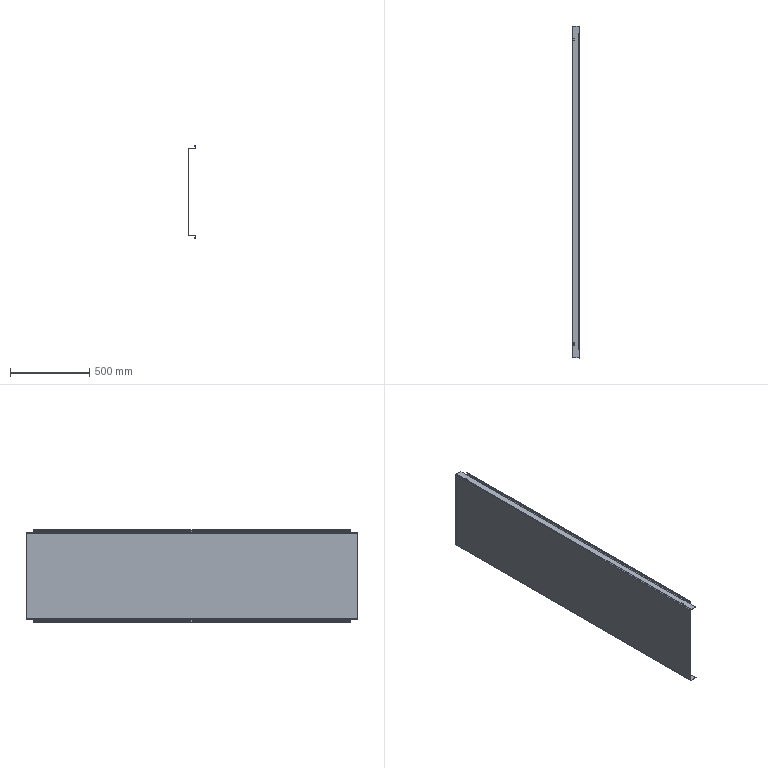Component | SolidWorks | Box-1 | 1 solid | 76 faces | volume 2872317 mm3 | plane 48 | cylinder 28 | commonest cylinder face diameters 4.5 x16 11 x6 7 x6 | material Plain Carbon Steel